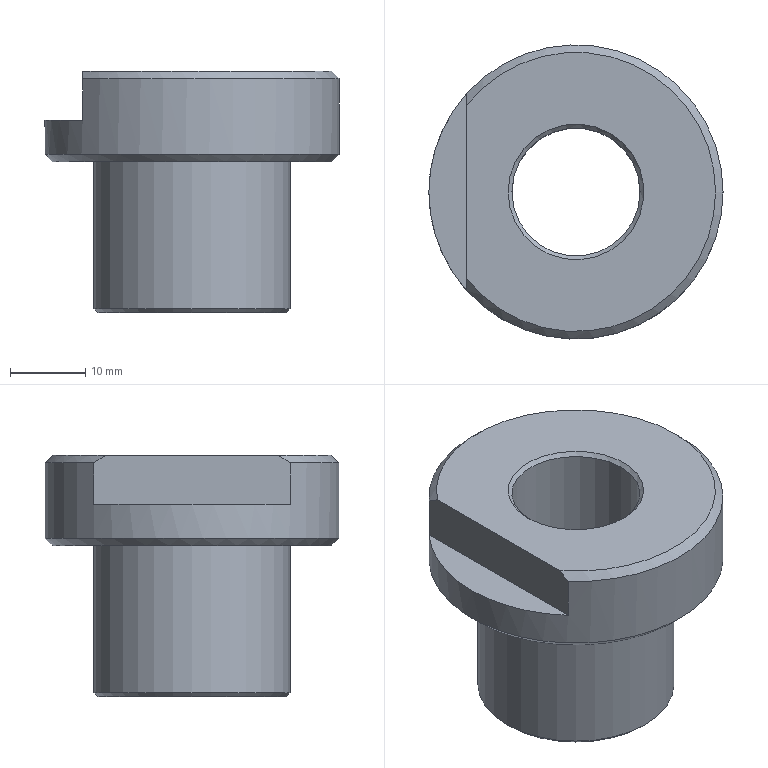Component | NX | DRILL_BUSH_2 | 1 solid | 13 faces | box 39 x 39 x 32 mm | volume 16979 mm3 | plane 5 | cone 5 | cylinder 3 | commonest cylinder face diameters 26 x1 39 x1 17 x1
STEP:
#1=CARTESIAN_POINT('',(0.,0.,0.));
#2=DIRECTION('',(0.,0.,1.));
#3=DIRECTION('',(1.,0.,0.));
#4=AXIS2_PLACEMENT_3D('',#1,#2,#3);
#5=CARTESIAN_POINT('',(99.,0.,190.));
#6=VERTEX_POINT('',#5);
#7=CARTESIAN_POINT('',(90.,0.,190.));
#8=DIRECTION('',(0.,0.,1.));
#9=DIRECTION('',(1.,0.,0.));
#10=AXIS2_PLACEMENT_3D('',#7,#8,#9);
#11=CIRCLE('',#10,9.);
#12=CARTESIAN_POINT('',(90.,0.,190.));
#13=DIRECTION('',(0.,0.,-1.));
#14=DIRECTION('',(1.,0.,0.));
#15=AXIS2_PLACEMENT_3D('',#12,#13,#14);
#16=PLANE('',#15);
#17=CARTESIAN_POINT('',(9.,0.));
#18=CARTESIAN_POINT('',(9.,-15.588));
#19=CARTESIAN_POINT('',(-4.5,-7.794));
#20=CARTESIAN_POINT('',(-18.,-0.));
#21=CARTESIAN_POINT('',(-4.5,7.794));
#22=CARTESIAN_POINT('',(9.,15.588));
#23=CARTESIAN_POINT('',(9.,0.));
#24=(BOUNDED_CURVE()B_SPLINE_CURVE(2,(#17,#18,#19,#20,#21,#22,#23),.UNSPECIFIED.,.T.,.F.)B_SPLINE_CURVE_WITH_KNOTS((1,2,2,2,2,1),(-2.094,0.,2.094,4.189,6.283,8.378),.UNSPECIFIED.)CURVE()GEOMETRIC_REPRESENTATION_ITEM()RATIONAL_B_SPLINE_CURVE((1.,0.5,1.,0.5,1.,0.5,1.))REPRESENTATION_ITEM(''));
#25=(GEOMETRIC_REPRESENTATION_CONTEXT(2)PARAMETRIC_REPRESENTATION_CONTEXT()REPRESENTATION_CONTEXT('',''));
#26=DEFINITIONAL_REPRESENTATION('',(#24),#25);
#27=PCURVE('',#16,#26);
#28=CARTESIAN_POINT('',(90.,0.,190.5));
#29=DIRECTION('',(0.,0.,-1.));
#30=DIRECTION('',(1.,0.,0.));
#31=AXIS2_PLACEMENT_3D('',#28,#29,#30);
#32=CONICAL_SURFACE('',#31,8.5,0.7854);
#33=CARTESIAN_POINT('',(6.283,0.5));
#34=DIRECTION('',(-1.,0.));
#35=VECTOR('',#34,1.);
#36=LINE('',#33,#35);
#37=(GEOMETRIC_REPRESENTATION_CONTEXT(2)PARAMETRIC_REPRESENTATION_CONTEXT()REPRESENTATION_CONTEXT('',''));
#38=DEFINITIONAL_REPRESENTATION('',(#36),#37);
#39=PCURVE('',#32,#38);
#40=SURFACE_CURVE('',#11,(#27,#39),.PCURVE_S1.);
#41=EDGE_CURVE('',#6,#6,#40,.T.);
#42=ORIENTED_EDGE('',*,*,#41,.T.);
#43=EDGE_LOOP('',(#42));
#44=FACE_BOUND('',#43,.T.);
#45=CARTESIAN_POINT('',(102.5,0.,190.));
#46=VERTEX_POINT('',#45);
#47=CARTESIAN_POINT('',(90.,0.,190.));
#48=DIRECTION('',(0.,0.,-1.));
#49=DIRECTION('',(1.,0.,0.));
#50=AXIS2_PLACEMENT_3D('',#47,#48,#49);
#51=CIRCLE('',#50,12.5);
#52=CARTESIAN_POINT('',(0.,0.));
#53=DIRECTION('',(1.,0.));
#54=AXIS2_PLACEMENT_2D('',#52,#53);
#55=CIRCLE('',#54,12.5);
#56=(GEOMETRIC_REPRESENTATION_CONTEXT(2)PARAMETRIC_REPRESENTATION_CONTEXT()REPRESENTATION_CONTEXT('',''));
#57=DEFINITIONAL_REPRESENTATION('',(#55),#56);
#58=PCURVE('',#16,#57);
#59=CARTESIAN_POINT('',(90.,0.,190.5));
#60=DIRECTION('',(0.,0.,1.));
#61=DIRECTION('',(-1.,0.,0.));
#62=AXIS2_PLACEMENT_3D('',#59,#60,#61);
#63=CONICAL_SURFACE('',#62,13.,0.7854);
#64=CARTESIAN_POINT('',(9.425,-0.5));
#65=DIRECTION('',(-1.,0.));
#66=VECTOR('',#65,1.);
#67=LINE('',#64,#66);
#68=(GEOMETRIC_REPRESENTATION_CONTEXT(2)PARAMETRIC_REPRESENTATION_CONTEXT()REPRESENTATION_CONTEXT('',''));
#69=DEFINITIONAL_REPRESENTATION('',(#67),#68);
#70=PCURVE('',#63,#69);
#71=SURFACE_CURVE('',#51,(#58,#70),.PCURVE_S1.);
#72=EDGE_CURVE('',#46,#46,#71,.T.);
#73=ORIENTED_EDGE('',*,*,#72,.T.);
#74=EDGE_LOOP('',(#73));
#75=FACE_BOUND('',#74,.T.);
#76=ADVANCED_FACE('',(#44,#75),#16,.T.);
#77=CARTESIAN_POINT('',(103.,0.,190.5));
#78=VERTEX_POINT('',#77);
#79=CARTESIAN_POINT('',(90.,0.,190.5));
#80=DIRECTION('',(0.,0.,1.));
#81=DIRECTION('',(1.,0.,0.));
#82=AXIS2_PLACEMENT_3D('',#79,#80,#81);
#83=CIRCLE('',#82,13.);
#84=CARTESIAN_POINT('',(90.,0.,190.));
#85=DIRECTION('',(0.,0.,1.));
#86=DIRECTION('',(-1.,0.,0.));
#87=AXIS2_PLACEMENT_3D('',#84,#85,#86);
#88=CYLINDRICAL_SURFACE('',#87,13.);
#89=CARTESIAN_POINT('',(3.142,0.5));
#90=DIRECTION('',(1.,0.));
#91=VECTOR('',#90,1.);
#92=LINE('',#89,#91);
#93=(GEOMETRIC_REPRESENTATION_CONTEXT(2)PARAMETRIC_REPRESENTATION_CONTEXT()REPRESENTATION_CONTEXT('',''));
#94=DEFINITIONAL_REPRESENTATION('',(#92),#93);
#95=PCURVE('',#88,#94);
#96=CARTESIAN_POINT('',(3.142,0.));
#97=DIRECTION('',(1.,0.));
#98=VECTOR('',#97,1.);
#99=LINE('',#96,#98);
#100=(GEOMETRIC_REPRESENTATION_CONTEXT(2)PARAMETRIC_REPRESENTATION_CONTEXT()REPRESENTATION_CONTEXT('',''));
#101=DEFINITIONAL_REPRESENTATION('',(#99),#100);
#102=PCURVE('',#63,#101);
#103=SURFACE_CURVE('',#83,(#95,#102),.PCURVE_S1.);
#104=EDGE_CURVE('',#78,#78,#103,.T.);
#105=ORIENTED_EDGE('',*,*,#104,.T.);
#106=CARTESIAN_POINT('',(103.,0.,210.));
#107=VERTEX_POINT('',#106);
#108=CARTESIAN_POINT('',(103.,0.,190.5));
#109=CARTESIAN_POINT('',(103.,0.,210.));
#110=B_SPLINE_CURVE_WITH_KNOTS('',1,(#108,#109),.UNSPECIFIED.,.F.,.F.,(2,2),(0.5,20.),.PIECEWISE_BEZIER_KNOTS.);
#111=CARTESIAN_POINT('',(9.425,0.));
#112=DIRECTION('',(0.,1.));
#113=VECTOR('',#112,1.);
#114=LINE('',#111,#113);
#115=(GEOMETRIC_REPRESENTATION_CONTEXT(2)PARAMETRIC_REPRESENTATION_CONTEXT()REPRESENTATION_CONTEXT('',''));
#116=DEFINITIONAL_REPRESENTATION('',(#114),#115);
#117=PCURVE('',#88,#116);
#118=CARTESIAN_POINT('',(3.142,0.));
#119=DIRECTION('',(0.,1.));
#120=VECTOR('',#119,1.);
#121=LINE('',#118,#120);
#122=(GEOMETRIC_REPRESENTATION_CONTEXT(2)PARAMETRIC_REPRESENTATION_CONTEXT()REPRESENTATION_CONTEXT('',''));
#123=DEFINITIONAL_REPRESENTATION('',(#121),#122);
#124=PCURVE('',#88,#123);
#125=SEAM_CURVE('',#110,(#117,#124),.PCURVE_S1.);
#126=EDGE_CURVE('',#78,#107,#125,.T.);
#127=ORIENTED_EDGE('',*,*,#126,.T.);
#128=CARTESIAN_POINT('',(90.,0.,210.));
#129=DIRECTION('',(0.,0.,1.));
#130=DIRECTION('',(1.,0.,0.));
#131=AXIS2_PLACEMENT_3D('',#128,#129,#130);
#132=CIRCLE('',#131,13.);
#133=CARTESIAN_POINT('',(3.142,20.));
#134=DIRECTION('',(1.,0.));
#135=VECTOR('',#134,1.);
#136=LINE('',#133,#135);
#137=(GEOMETRIC_REPRESENTATION_CONTEXT(2)PARAMETRIC_REPRESENTATION_CONTEXT()REPRESENTATION_CONTEXT('',''));
#138=DEFINITIONAL_REPRESENTATION('',(#136),#137);
#139=PCURVE('',#88,#138);
#140=CARTESIAN_POINT('',(90.,0.,210.));
#141=DIRECTION('',(0.,0.,-1.));
#142=DIRECTION('',(1.,0.,0.));
#143=AXIS2_PLACEMENT_3D('',#140,#141,#142);
#144=PLANE('',#143);
#145=CARTESIAN_POINT('',(13.,0.));
#146=CARTESIAN_POINT('',(13.,-22.517));
#147=CARTESIAN_POINT('',(-6.5,-11.258));
#148=CARTESIAN_POINT('',(-26.,-0.));
#149=CARTESIAN_POINT('',(-6.5,11.258));
#150=CARTESIAN_POINT('',(13.,22.517));
#151=CARTESIAN_POINT('',(13.,0.));
#152=(BOUNDED_CURVE()B_SPLINE_CURVE(2,(#145,#146,#147,#148,#149,#150,#151),.UNSPECIFIED.,.T.,.F.)B_SPLINE_CURVE_WITH_KNOTS((1,2,2,2,2,1),(-2.094,0.,2.094,4.189,6.283,8.378),.UNSPECIFIED.)CURVE()GEOMETRIC_REPRESENTATION_ITEM()RATIONAL_B_SPLINE_CURVE((1.,0.5,1.,0.5,1.,0.5,1.))REPRESENTATION_ITEM(''));
#153=(GEOMETRIC_REPRESENTATION_CONTEXT(2)PARAMETRIC_REPRESENTATION_CONTEXT()REPRESENTATION_CONTEXT('',''));
#154=DEFINITIONAL_REPRESENTATION('',(#152),#153);
#155=PCURVE('',#144,#154);
#156=SURFACE_CURVE('',#132,(#139,#155),.PCURVE_S1.);
#157=EDGE_CURVE('',#107,#107,#156,.T.);
#158=ORIENTED_EDGE('',*,*,#157,.F.);
#159=ORIENTED_EDGE('',*,*,#126,.F.);
#160=EDGE_LOOP('',(#105,#127,#158,#159));
#161=FACE_BOUND('',#160,.T.);
#162=ADVANCED_FACE('',(#161),#88,.T.);
#163=CARTESIAN_POINT('',(81.,0.,222.));
#164=VERTEX_POINT('',#163);
#165=CARTESIAN_POINT('',(90.,0.,222.));
#166=DIRECTION('',(0.,0.,-1.));
#167=DIRECTION('',(-1.,0.,0.));
#168=AXIS2_PLACEMENT_3D('',#165,#166,#167);
#169=CIRCLE('',#168,9.);
#170=CARTESIAN_POINT('',(90.,0.,222.));
#171=DIRECTION('',(0.,0.,1.));
#172=DIRECTION('',(-1.,0.,0.));
#173=AXIS2_PLACEMENT_3D('',#170,#171,#172);
#174=PLANE('',#173);
#175=CARTESIAN_POINT('',(9.,0.));
#176=CARTESIAN_POINT('',(9.,-15.588));
#177=CARTESIAN_POINT('',(-4.5,-7.794));
#178=CARTESIAN_POINT('',(-18.,-0.));
#179=CARTESIAN_POINT('',(-4.5,7.794));
#180=CARTESIAN_POINT('',(9.,15.588));
#181=CARTESIAN_POINT('',(9.,0.));
#182=(BOUNDED_CURVE()B_SPLINE_CURVE(2,(#175,#176,#177,#178,#179,#180,#181),.UNSPECIFIED.,.T.,.F.)B_SPLINE_CURVE_WITH_KNOTS((1,2,2,2,2,1),(-2.094,0.,2.094,4.189,6.283,8.378),.UNSPECIFIED.)CURVE()GEOMETRIC_REPRESENTATION_ITEM()RATIONAL_B_SPLINE_CURVE((1.,0.5,1.,0.5,1.,0.5,1.))REPRESENTATION_ITEM(''));
#183=(GEOMETRIC_REPRESENTATION_CONTEXT(2)PARAMETRIC_REPRESENTATION_CONTEXT()REPRESENTATION_CONTEXT('',''));
#184=DEFINITIONAL_REPRESENTATION('',(#182),#183);
#185=PCURVE('',#174,#184);
#186=CARTESIAN_POINT('',(90.,0.,222.));
#187=DIRECTION('',(0.,0.,1.));
#188=DIRECTION('',(-1.,0.,0.));
#189=AXIS2_PLACEMENT_3D('',#186,#187,#188);
#190=CONICAL_SURFACE('',#189,9.,0.7854);
#191=CARTESIAN_POINT('',(6.283,0.));
#192=DIRECTION('',(-1.,0.));
#193=VECTOR('',#192,1.);
#194=LINE('',#191,#193);
#195=(GEOMETRIC_REPRESENTATION_CONTEXT(2)PARAMETRIC_REPRESENTATION_CONTEXT()REPRESENTATION_CONTEXT('',''));
#196=DEFINITIONAL_REPRESENTATION('',(#194),#195);
#197=PCURVE('',#190,#196);
#198=SURFACE_CURVE('',#169,(#185,#197),.PCURVE_S1.);
#199=EDGE_CURVE('',#164,#164,#198,.T.);
#200=ORIENTED_EDGE('',*,*,#199,.T.);
#201=EDGE_LOOP('',(#200));
#202=FACE_BOUND('',#201,.T.);
#203=CARTESIAN_POINT('',(75.5,-11.489,222.));
#204=VERTEX_POINT('',#203);
#205=CARTESIAN_POINT('',(75.5,11.489,222.));
#206=VERTEX_POINT('',#205);
#207=CARTESIAN_POINT('',(75.5,-22.5,222.));
#208=DIRECTION('',(-0.,1.,0.));
#209=VECTOR('',#208,1.);
#210=LINE('',#207,#209);
#211=CARTESIAN_POINT('',(14.5,22.5));
#212=DIRECTION('',(0.,-1.));
#213=VECTOR('',#212,1.);
#214=LINE('',#211,#213);
#215=(GEOMETRIC_REPRESENTATION_CONTEXT(2)PARAMETRIC_REPRESENTATION_CONTEXT()REPRESENTATION_CONTEXT('',''));
#216=DEFINITIONAL_REPRESENTATION('',(#214),#215);
#217=PCURVE('',#174,#216);
#218=CARTESIAN_POINT('',(75.5,-22.5,215.5));
#219=DIRECTION('',(1.,0.,0.));
#220=DIRECTION('',(-0.,1.,0.));
#221=AXIS2_PLACEMENT_3D('',#218,#219,#220);
#222=PLANE('',#221);
#223=CARTESIAN_POINT('',(0.,6.5));
#224=DIRECTION('',(1.,0.));
#225=VECTOR('',#224,1.);
#226=LINE('',#223,#225);
#227=(GEOMETRIC_REPRESENTATION_CONTEXT(2)PARAMETRIC_REPRESENTATION_CONTEXT()REPRESENTATION_CONTEXT('',''));
#228=DEFINITIONAL_REPRESENTATION('',(#226),#227);
#229=PCURVE('',#222,#228);
#230=SURFACE_CURVE('',#210,(#217,#229),.PCURVE_S1.);
#231=EDGE_CURVE('',#204,#206,#230,.T.);
#232=ORIENTED_EDGE('',*,*,#231,.F.);
#233=CARTESIAN_POINT('',(90.,0.,222.));
#234=DIRECTION('',(0.,0.,1.));
#235=DIRECTION('',(-1.,0.,0.));
#236=AXIS2_PLACEMENT_3D('',#233,#234,#235);
#237=CIRCLE('',#236,18.5);
#238=CARTESIAN_POINT('',(0.,0.));
#239=DIRECTION('',(1.,0.));
#240=AXIS2_PLACEMENT_2D('',#238,#239);
#241=CIRCLE('',#240,18.5);
#242=(GEOMETRIC_REPRESENTATION_CONTEXT(2)PARAMETRIC_REPRESENTATION_CONTEXT()REPRESENTATION_CONTEXT('',''));
#243=DEFINITIONAL_REPRESENTATION('',(#241),#242);
#244=PCURVE('',#174,#243);
#245=CARTESIAN_POINT('',(90.,0.,221.));
#246=DIRECTION('',(0.,0.,-1.));
#247=DIRECTION('',(1.,0.,0.));
#248=AXIS2_PLACEMENT_3D('',#245,#246,#247);
#249=CONICAL_SURFACE('',#248,19.5,0.7854);
#250=CARTESIAN_POINT('',(3.142,-1.));
#251=DIRECTION('',(-1.,-0.));
#252=VECTOR('',#251,1.);
#253=LINE('',#250,#252);
#254=(GEOMETRIC_REPRESENTATION_CONTEXT(2)PARAMETRIC_REPRESENTATION_CONTEXT()REPRESENTATION_CONTEXT('',''));
#255=DEFINITIONAL_REPRESENTATION('',(#253),#254);
#256=PCURVE('',#249,#255);
#257=SURFACE_CURVE('',#237,(#244,#256),.PCURVE_S1.);
#258=EDGE_CURVE('',#204,#206,#257,.T.);
#259=ORIENTED_EDGE('',*,*,#258,.T.);
#260=EDGE_LOOP('',(#232,#259));
#261=FACE_BOUND('',#260,.T.);
#262=ADVANCED_FACE('',(#202,#261),#174,.T.);
#263=CARTESIAN_POINT('',(108.5,0.,210.));
#264=VERTEX_POINT('',#263);
#265=CARTESIAN_POINT('',(90.,0.,210.));
#266=DIRECTION('',(0.,0.,-1.));
#267=DIRECTION('',(1.,0.,0.));
#268=AXIS2_PLACEMENT_3D('',#265,#266,#267);
#269=CIRCLE('',#268,18.5);
#270=CARTESIAN_POINT('',(0.,0.));
#271=DIRECTION('',(1.,0.));
#272=AXIS2_PLACEMENT_2D('',#270,#271);
#273=CIRCLE('',#272,18.5);
#274=(GEOMETRIC_REPRESENTATION_CONTEXT(2)PARAMETRIC_REPRESENTATION_CONTEXT()REPRESENTATION_CONTEXT('',''));
#275=DEFINITIONAL_REPRESENTATION('',(#273),#274);
#276=PCURVE('',#144,#275);
#277=CARTESIAN_POINT('',(90.,0.,211.));
#278=DIRECTION('',(0.,0.,1.));
#279=DIRECTION('',(-1.,0.,0.));
#280=AXIS2_PLACEMENT_3D('',#277,#278,#279);
#281=CONICAL_SURFACE('',#280,19.5,0.7854);
#282=CARTESIAN_POINT('',(9.425,-1.));
#283=DIRECTION('',(-1.,0.));
#284=VECTOR('',#283,1.);
#285=LINE('',#282,#284);
#286=(GEOMETRIC_REPRESENTATION_CONTEXT(2)PARAMETRIC_REPRESENTATION_CONTEXT()REPRESENTATION_CONTEXT('',''));
#287=DEFINITIONAL_REPRESENTATION('',(#285),#286);
#288=PCURVE('',#281,#287);
#289=SURFACE_CURVE('',#269,(#276,#288),.PCURVE_S1.);
#290=EDGE_CURVE('',#264,#264,#289,.T.);
#291=ORIENTED_EDGE('',*,*,#290,.T.);
#292=EDGE_LOOP('',(#291));
#293=FACE_BOUND('',#292,.T.);
#294=ORIENTED_EDGE('',*,*,#157,.T.);
#295=EDGE_LOOP('',(#294));
#296=FACE_BOUND('',#295,.T.);
#297=ADVANCED_FACE('',(#293,#296),#144,.T.);
#298=CARTESIAN_POINT('',(109.5,0.,211.));
#299=VERTEX_POINT('',#298);
#300=CARTESIAN_POINT('',(75.5,13.038,211.));
#301=VERTEX_POINT('',#300);
#302=CARTESIAN_POINT('',(90.,0.,211.));
#303=DIRECTION('',(0.,0.,1.));
#304=DIRECTION('',(1.,0.,0.));
#305=AXIS2_PLACEMENT_3D('',#302,#303,#304);
#306=CIRCLE('',#305,19.5);
#307=CARTESIAN_POINT('',(90.,0.,210.));
#308=DIRECTION('',(0.,0.,1.));
#309=DIRECTION('',(-1.,0.,0.));
#310=AXIS2_PLACEMENT_3D('',#307,#308,#309);
#311=CYLINDRICAL_SURFACE('',#310,19.5);
#312=CARTESIAN_POINT('',(9.425,1.));
#313=DIRECTION('',(1.,0.));
#314=VECTOR('',#313,1.);
#315=LINE('',#312,#314);
#316=(GEOMETRIC_REPRESENTATION_CONTEXT(2)PARAMETRIC_REPRESENTATION_CONTEXT()REPRESENTATION_CONTEXT('',''));
#317=DEFINITIONAL_REPRESENTATION('',(#315),#316);
#318=PCURVE('',#311,#317);
#319=CARTESIAN_POINT('',(3.142,0.));
#320=DIRECTION('',(1.,0.));
#321=VECTOR('',#320,1.);
#322=LINE('',#319,#321);
#323=(GEOMETRIC_REPRESENTATION_CONTEXT(2)PARAMETRIC_REPRESENTATION_CONTEXT()REPRESENTATION_CONTEXT('',''));
#324=DEFINITIONAL_REPRESENTATION('',(#322),#323);
#325=PCURVE('',#281,#324);
#326=SURFACE_CURVE('',#306,(#318,#325),.PCURVE_S1.);
#327=EDGE_CURVE('',#299,#301,#326,.T.);
#328=ORIENTED_EDGE('',*,*,#327,.T.);
#329=CARTESIAN_POINT('',(75.5,13.038,215.5));
#330=VERTEX_POINT('',#329);
#331=CARTESIAN_POINT('',(75.5,13.038,211.));
#332=CARTESIAN_POINT('',(75.5,13.038,215.5));
#333=B_SPLINE_CURVE_WITH_KNOTS('',1,(#331,#332),.UNSPECIFIED.,.F.,.F.,(2,2),(1.,5.5),.PIECEWISE_BEZIER_KNOTS.);
#334=CARTESIAN_POINT('',(11.834,0.));
#335=DIRECTION('',(0.,1.));
#336=VECTOR('',#335,1.);
#337=LINE('',#334,#336);
#338=(GEOMETRIC_REPRESENTATION_CONTEXT(2)PARAMETRIC_REPRESENTATION_CONTEXT()REPRESENTATION_CONTEXT('',''));
#339=DEFINITIONAL_REPRESENTATION('',(#337),#338);
#340=PCURVE('',#311,#339);
#341=CARTESIAN_POINT('',(5.551,0.));
#342=DIRECTION('',(0.,1.));
#343=VECTOR('',#342,1.);
#344=LINE('',#341,#343);
#345=(GEOMETRIC_REPRESENTATION_CONTEXT(2)PARAMETRIC_REPRESENTATION_CONTEXT()REPRESENTATION_CONTEXT('',''));
#346=DEFINITIONAL_REPRESENTATION('',(#344),#345);
#347=PCURVE('',#311,#346);
#348=SEAM_CURVE('',#333,(#340,#347),.PCURVE_S1.);
#349=EDGE_CURVE('',#301,#330,#348,.T.);
#350=ORIENTED_EDGE('',*,*,#349,.T.);
#351=CARTESIAN_POINT('',(75.5,13.038,221.));
#352=VERTEX_POINT('',#351);
#353=CARTESIAN_POINT('',(75.5,13.038,210.));
#354=DIRECTION('',(0.,0.,-1.));
#355=VECTOR('',#354,1.);
#356=LINE('',#353,#355);
#357=CARTESIAN_POINT('',(11.834,0.));
#358=DIRECTION('',(0.,-1.));
#359=VECTOR('',#358,1.);
#360=LINE('',#357,#359);
#361=(GEOMETRIC_REPRESENTATION_CONTEXT(2)PARAMETRIC_REPRESENTATION_CONTEXT()REPRESENTATION_CONTEXT('',''));
#362=DEFINITIONAL_REPRESENTATION('',(#360),#361);
#363=PCURVE('',#311,#362);
#364=CARTESIAN_POINT('',(35.538,-5.5));
#365=DIRECTION('',(0.,-1.));
#366=VECTOR('',#365,1.);
#367=LINE('',#364,#366);
#368=(GEOMETRIC_REPRESENTATION_CONTEXT(2)PARAMETRIC_REPRESENTATION_CONTEXT()REPRESENTATION_CONTEXT('',''));
#369=DEFINITIONAL_REPRESENTATION('',(#367),#368);
#370=PCURVE('',#222,#369);
#371=SURFACE_CURVE('',#356,(#363,#370),.PCURVE_S1.);
#372=EDGE_CURVE('',#352,#330,#371,.T.);
#373=ORIENTED_EDGE('',*,*,#372,.F.);
#374=CARTESIAN_POINT('',(75.5,-13.038,221.));
#375=VERTEX_POINT('',#374);
#376=CARTESIAN_POINT('',(90.,0.,221.));
#377=DIRECTION('',(0.,0.,-1.));
#378=DIRECTION('',(-1.,0.,0.));
#379=AXIS2_PLACEMENT_3D('',#376,#377,#378);
#380=CIRCLE('',#379,19.5);
#381=CARTESIAN_POINT('',(12.566,11.));
#382=DIRECTION('',(-1.,0.));
#383=VECTOR('',#382,1.);
#384=LINE('',#381,#383);
#385=(GEOMETRIC_REPRESENTATION_CONTEXT(2)PARAMETRIC_REPRESENTATION_CONTEXT()REPRESENTATION_CONTEXT('',''));
#386=DEFINITIONAL_REPRESENTATION('',(#384),#385);
#387=PCURVE('',#311,#386);
#388=CARTESIAN_POINT('',(-3.142,-0.));
#389=DIRECTION('',(1.,0.));
#390=VECTOR('',#389,1.);
#391=LINE('',#388,#390);
#392=(GEOMETRIC_REPRESENTATION_CONTEXT(2)PARAMETRIC_REPRESENTATION_CONTEXT()REPRESENTATION_CONTEXT('',''));
#393=DEFINITIONAL_REPRESENTATION('',(#391),#392);
#394=PCURVE('',#249,#393);
#395=SURFACE_CURVE('',#380,(#387,#394),.PCURVE_S1.);
#396=EDGE_CURVE('',#352,#375,#395,.T.);
#397=ORIENTED_EDGE('',*,*,#396,.T.);
#398=CARTESIAN_POINT('',(75.5,-13.038,215.5));
#399=VERTEX_POINT('',#398);
#400=CARTESIAN_POINT('',(75.5,-13.038,210.));
#401=DIRECTION('',(0.,0.,1.));
#402=VECTOR('',#401,1.);
#403=LINE('',#400,#402);
#404=CARTESIAN_POINT('',(7.016,0.));
#405=DIRECTION('',(0.,1.));
#406=VECTOR('',#405,1.);
#407=LINE('',#404,#406);
#408=(GEOMETRIC_REPRESENTATION_CONTEXT(2)PARAMETRIC_REPRESENTATION_CONTEXT()REPRESENTATION_CONTEXT('',''));
#409=DEFINITIONAL_REPRESENTATION('',(#407),#408);
#410=PCURVE('',#311,#409);
#411=CARTESIAN_POINT('',(9.462,-5.5));
#412=DIRECTION('',(0.,1.));
#413=VECTOR('',#412,1.);
#414=LINE('',#411,#413);
#415=(GEOMETRIC_REPRESENTATION_CONTEXT(2)PARAMETRIC_REPRESENTATION_CONTEXT()REPRESENTATION_CONTEXT('',''));
#416=DEFINITIONAL_REPRESENTATION('',(#414),#415);
#417=PCURVE('',#222,#416);
#418=SURFACE_CURVE('',#403,(#410,#417),.PCURVE_S1.);
#419=EDGE_CURVE('',#399,#375,#418,.T.);
#420=ORIENTED_EDGE('',*,*,#419,.F.);
#421=CARTESIAN_POINT('',(90.,0.,215.5));
#422=DIRECTION('',(0.,0.,-1.));
#423=DIRECTION('',(-1.,0.,0.));
#424=AXIS2_PLACEMENT_3D('',#421,#422,#423);
#425=CIRCLE('',#424,19.5);
#426=CARTESIAN_POINT('',(12.566,5.5));
#427=DIRECTION('',(-1.,0.));
#428=VECTOR('',#427,1.);
#429=LINE('',#426,#428);
#430=(GEOMETRIC_REPRESENTATION_CONTEXT(2)PARAMETRIC_REPRESENTATION_CONTEXT()REPRESENTATION_CONTEXT('',''));
#431=DEFINITIONAL_REPRESENTATION('',(#429),#430);
#432=PCURVE('',#311,#431);
#433=CARTESIAN_POINT('',(90.,0.,215.5));
#434=DIRECTION('',(0.,0.,1.));
#435=DIRECTION('',(-1.,0.,0.));
#436=AXIS2_PLACEMENT_3D('',#433,#434,#435);
#437=PLANE('',#436);
#438=CARTESIAN_POINT('',(19.5,0.));
#439=CARTESIAN_POINT('',(19.5,-33.775));
#440=CARTESIAN_POINT('',(-9.75,-16.887));
#441=CARTESIAN_POINT('',(-39.,-0.));
#442=CARTESIAN_POINT('',(-9.75,16.887));
#443=CARTESIAN_POINT('',(19.5,33.775));
#444=CARTESIAN_POINT('',(19.5,0.));
#445=(BOUNDED_CURVE()B_SPLINE_CURVE(2,(#438,#439,#440,#441,#442,#443,#444),.UNSPECIFIED.,.T.,.F.)B_SPLINE_CURVE_WITH_KNOTS((1,2,2,2,2,1),(-2.094,0.,2.094,4.189,6.283,8.378),.UNSPECIFIED.)CURVE()GEOMETRIC_REPRESENTATION_ITEM()RATIONAL_B_SPLINE_CURVE((1.,0.5,1.,0.5,1.,0.5,1.))REPRESENTATION_ITEM(''));
#446=(GEOMETRIC_REPRESENTATION_CONTEXT(2)PARAMETRIC_REPRESENTATION_CONTEXT()REPRESENTATION_CONTEXT('',''));
#447=DEFINITIONAL_REPRESENTATION('',(#445),#446);
#448=PCURVE('',#437,#447);
#449=SURFACE_CURVE('',#425,(#432,#448),.PCURVE_S1.);
#450=EDGE_CURVE('',#399,#330,#449,.T.);
#451=ORIENTED_EDGE('',*,*,#450,.T.);
#452=ORIENTED_EDGE('',*,*,#349,.F.);
#453=CARTESIAN_POINT('',(90.,0.,211.));
#454=DIRECTION('',(0.,0.,1.));
#455=DIRECTION('',(1.,0.,0.));
#456=AXIS2_PLACEMENT_3D('',#453,#454,#455);
#457=CIRCLE('',#456,19.5);
#458=CARTESIAN_POINT('',(3.142,1.));
#459=DIRECTION('',(1.,0.));
#460=VECTOR('',#459,1.);
#461=LINE('',#458,#460);
#462=(GEOMETRIC_REPRESENTATION_CONTEXT(2)PARAMETRIC_REPRESENTATION_CONTEXT()REPRESENTATION_CONTEXT('',''));
#463=DEFINITIONAL_REPRESENTATION('',(#461),#462);
#464=PCURVE('',#311,#463);
#465=CARTESIAN_POINT('',(3.142,0.));
#466=DIRECTION('',(1.,0.));
#467=VECTOR('',#466,1.);
#468=LINE('',#465,#467);
#469=(GEOMETRIC_REPRESENTATION_CONTEXT(2)PARAMETRIC_REPRESENTATION_CONTEXT()REPRESENTATION_CONTEXT('',''));
#470=DEFINITIONAL_REPRESENTATION('',(#468),#469);
#471=PCURVE('',#281,#470);
#472=SURFACE_CURVE('',#457,(#464,#471),.PCURVE_S1.);
#473=EDGE_CURVE('',#301,#299,#472,.T.);
#474=ORIENTED_EDGE('',*,*,#473,.T.);
#475=EDGE_LOOP('',(#328,#350,#373,#397,#420,#451,#452,#474));
#476=FACE_BOUND('',#475,.T.);
#477=ADVANCED_FACE('',(#476),#311,.T.);
#478=ORIENTED_EDGE('',*,*,#419,.T.);
#479=CARTESIAN_POINT('',(75.5,-13.038,221.));
#480=CARTESIAN_POINT('',(75.5,-12.527,221.342));
#481=CARTESIAN_POINT('',(75.5,-12.011,221.676));
#482=CARTESIAN_POINT('',(75.5,-11.489,222.));
#483=B_SPLINE_CURVE_WITH_KNOTS('',3,(#479,#480,#481,#482),.UNSPECIFIED.,.F.,.F.,(4,4),(0.,1.),.PIECEWISE_BEZIER_KNOTS.);
#484=CARTESIAN_POINT('',(9.462,5.5));
#485=CARTESIAN_POINT('',(9.973,5.842));
#486=CARTESIAN_POINT('',(10.489,6.176));
#487=CARTESIAN_POINT('',(11.011,6.5));
#488=B_SPLINE_CURVE_WITH_KNOTS('',3,(#484,#485,#486,#487),.UNSPECIFIED.,.F.,.F.,(4,4),(0.,1.),.PIECEWISE_BEZIER_KNOTS.);
#489=(GEOMETRIC_REPRESENTATION_CONTEXT(2)PARAMETRIC_REPRESENTATION_CONTEXT()REPRESENTATION_CONTEXT('',''));
#490=DEFINITIONAL_REPRESENTATION('',(#488),#489);
#491=PCURVE('',#222,#490);
#492=CARTESIAN_POINT('',(2.409,0.));
#493=CARTESIAN_POINT('',(2.472,-1.));
#494=B_SPLINE_CURVE_WITH_KNOTS('',1,(#492,#493),.UNSPECIFIED.,.F.,.F.,(2,2),(0.,1.),.PIECEWISE_BEZIER_KNOTS.);
#495=(GEOMETRIC_REPRESENTATION_CONTEXT(2)PARAMETRIC_REPRESENTATION_CONTEXT()REPRESENTATION_CONTEXT('',''));
#496=DEFINITIONAL_REPRESENTATION('',(#494),#495);
#497=PCURVE('',#249,#496);
#498=SURFACE_CURVE('',#483,(#491,#497),.PCURVE_S1.);
#499=EDGE_CURVE('',#375,#204,#498,.T.);
#500=ORIENTED_EDGE('',*,*,#499,.T.);
#501=ORIENTED_EDGE('',*,*,#231,.T.);
#502=CARTESIAN_POINT('',(75.5,11.489,222.));
#503=CARTESIAN_POINT('',(75.5,12.011,221.676));
#504=CARTESIAN_POINT('',(75.5,12.527,221.342));
#505=CARTESIAN_POINT('',(75.5,13.038,221.));
#506=B_SPLINE_CURVE_WITH_KNOTS('',3,(#502,#503,#504,#505),.UNSPECIFIED.,.F.,.F.,(4,4),(0.,1.),.PIECEWISE_BEZIER_KNOTS.);
#507=CARTESIAN_POINT('',(33.989,6.5));
#508=CARTESIAN_POINT('',(34.511,6.176));
#509=CARTESIAN_POINT('',(35.027,5.842));
#510=CARTESIAN_POINT('',(35.538,5.5));
#511=B_SPLINE_CURVE_WITH_KNOTS('',3,(#507,#508,#509,#510),.UNSPECIFIED.,.F.,.F.,(4,4),(0.,1.),.PIECEWISE_BEZIER_KNOTS.);
#512=(GEOMETRIC_REPRESENTATION_CONTEXT(2)PARAMETRIC_REPRESENTATION_CONTEXT()REPRESENTATION_CONTEXT('',''));
#513=DEFINITIONAL_REPRESENTATION('',(#511),#512);
#514=PCURVE('',#222,#513);
#515=CARTESIAN_POINT('',(-2.472,-1.));
#516=CARTESIAN_POINT('',(-2.409,-0.));
#517=B_SPLINE_CURVE_WITH_KNOTS('',1,(#515,#516),.UNSPECIFIED.,.F.,.F.,(2,2),(0.,1.),.PIECEWISE_BEZIER_KNOTS.);
#518=(GEOMETRIC_REPRESENTATION_CONTEXT(2)PARAMETRIC_REPRESENTATION_CONTEXT()REPRESENTATION_CONTEXT('',''));
#519=DEFINITIONAL_REPRESENTATION('',(#517),#518);
#520=PCURVE('',#249,#519);
#521=SURFACE_CURVE('',#506,(#514,#520),.PCURVE_S1.);
#522=EDGE_CURVE('',#206,#352,#521,.T.);
#523=ORIENTED_EDGE('',*,*,#522,.T.);
#524=ORIENTED_EDGE('',*,*,#372,.T.);
#525=CARTESIAN_POINT('',(75.5,-22.5,215.5));
#526=DIRECTION('',(0.,-1.,0.));
#527=VECTOR('',#526,1.);
#528=LINE('',#525,#527);
#529=CARTESIAN_POINT('',(0.,0.));
#530=DIRECTION('',(-1.,0.));
#531=VECTOR('',#530,1.);
#532=LINE('',#529,#531);
#533=(GEOMETRIC_REPRESENTATION_CONTEXT(2)PARAMETRIC_REPRESENTATION_CONTEXT()REPRESENTATION_CONTEXT('',''));
#534=DEFINITIONAL_REPRESENTATION('',(#532),#533);
#535=PCURVE('',#222,#534);
#536=CARTESIAN_POINT('',(14.5,22.5));
#537=DIRECTION('',(-0.,1.));
#538=VECTOR('',#537,1.);
#539=LINE('',#536,#538);
#540=(GEOMETRIC_REPRESENTATION_CONTEXT(2)PARAMETRIC_REPRESENTATION_CONTEXT()REPRESENTATION_CONTEXT('',''));
#541=DEFINITIONAL_REPRESENTATION('',(#539),#540);
#542=PCURVE('',#437,#541);
#543=SURFACE_CURVE('',#528,(#535,#542),.PCURVE_S1.);
#544=EDGE_CURVE('',#330,#399,#543,.T.);
#545=ORIENTED_EDGE('',*,*,#544,.T.);
#546=EDGE_LOOP('',(#478,#500,#501,#523,#524,#545));
#547=FACE_BOUND('',#546,.T.);
#548=ADVANCED_FACE('',(#547),#222,.F.);
#549=ORIENTED_EDGE('',*,*,#544,.F.);
#550=ORIENTED_EDGE('',*,*,#450,.F.);
#551=EDGE_LOOP('',(#549,#550));
#552=FACE_BOUND('',#551,.T.);
#553=ADVANCED_FACE('',(#552),#437,.T.);
#554=CARTESIAN_POINT('',(98.5,0.,190.5));
#555=VERTEX_POINT('',#554);
#556=CARTESIAN_POINT('',(90.,0.,190.5));
#557=DIRECTION('',(0.,0.,-1.));
#558=DIRECTION('',(1.,0.,0.));
#559=AXIS2_PLACEMENT_3D('',#556,#557,#558);
#560=CIRCLE('',#559,8.5);
#561=CARTESIAN_POINT('',(90.,0.,222.));
#562=DIRECTION('',(0.,0.,-1.));
#563=DIRECTION('',(1.,0.,0.));
#564=AXIS2_PLACEMENT_3D('',#561,#562,#563);
#565=CYLINDRICAL_SURFACE('',#564,8.5);
#566=CARTESIAN_POINT('',(0.,31.5));
#567=DIRECTION('',(1.,0.));
#568=VECTOR('',#567,1.);
#569=LINE('',#566,#568);
#570=(GEOMETRIC_REPRESENTATION_CONTEXT(2)PARAMETRIC_REPRESENTATION_CONTEXT()REPRESENTATION_CONTEXT('',''));
#571=DEFINITIONAL_REPRESENTATION('',(#569),#570);
#572=PCURVE('',#565,#571);
#573=CARTESIAN_POINT('',(0.,0.));
#574=DIRECTION('',(1.,0.));
#575=VECTOR('',#574,1.);
#576=LINE('',#573,#575);
#577=(GEOMETRIC_REPRESENTATION_CONTEXT(2)PARAMETRIC_REPRESENTATION_CONTEXT()REPRESENTATION_CONTEXT('',''));
#578=DEFINITIONAL_REPRESENTATION('',(#576),#577);
#579=PCURVE('',#32,#578);
#580=SURFACE_CURVE('',#560,(#572,#579),.PCURVE_S1.);
#581=EDGE_CURVE('',#555,#555,#580,.T.);
#582=ORIENTED_EDGE('',*,*,#581,.F.);
#583=CARTESIAN_POINT('',(98.5,0.,221.5));
#584=VERTEX_POINT('',#583);
#585=CARTESIAN_POINT('',(98.5,0.,221.5));
#586=CARTESIAN_POINT('',(98.5,0.,190.5));
#587=B_SPLINE_CURVE_WITH_KNOTS('',1,(#585,#586),.UNSPECIFIED.,.F.,.F.,(2,2),(0.5,31.5),.PIECEWISE_BEZIER_KNOTS.);
#588=CARTESIAN_POINT('',(0.,0.));
#589=DIRECTION('',(0.,1.));
#590=VECTOR('',#589,1.);
#591=LINE('',#588,#590);
#592=(GEOMETRIC_REPRESENTATION_CONTEXT(2)PARAMETRIC_REPRESENTATION_CONTEXT()REPRESENTATION_CONTEXT('',''));
#593=DEFINITIONAL_REPRESENTATION('',(#591),#592);
#594=PCURVE('',#565,#593);
#595=CARTESIAN_POINT('',(6.283,0.));
#596=DIRECTION('',(0.,1.));
#597=VECTOR('',#596,1.);
#598=LINE('',#595,#597);
#599=(GEOMETRIC_REPRESENTATION_CONTEXT(2)PARAMETRIC_REPRESENTATION_CONTEXT()REPRESENTATION_CONTEXT('',''));
#600=DEFINITIONAL_REPRESENTATION('',(#598),#599);
#601=PCURVE('',#565,#600);
#602=SEAM_CURVE('',#587,(#594,#601),.PCURVE_S1.);
#603=EDGE_CURVE('',#584,#555,#602,.T.);
#604=ORIENTED_EDGE('',*,*,#603,.F.);
#605=CARTESIAN_POINT('',(81.5,0.,221.5));
#606=VERTEX_POINT('',#605);
#607=CARTESIAN_POINT('',(90.,0.,221.5));
#608=DIRECTION('',(0.,0.,1.));
#609=DIRECTION('',(-1.,0.,0.));
#610=AXIS2_PLACEMENT_3D('',#607,#608,#609);
#611=CIRCLE('',#610,8.5);
#612=CARTESIAN_POINT('',(3.142,0.5));
#613=DIRECTION('',(-1.,0.));
#614=VECTOR('',#613,1.);
#615=LINE('',#612,#614);
#616=(GEOMETRIC_REPRESENTATION_CONTEXT(2)PARAMETRIC_REPRESENTATION_CONTEXT()REPRESENTATION_CONTEXT('',''));
#617=DEFINITIONAL_REPRESENTATION('',(#615),#616);
#618=PCURVE('',#565,#617);
#619=CARTESIAN_POINT('',(0.,-0.5));
#620=DIRECTION('',(1.,0.));
#621=VECTOR('',#620,1.);
#622=LINE('',#619,#621);
#623=(GEOMETRIC_REPRESENTATION_CONTEXT(2)PARAMETRIC_REPRESENTATION_CONTEXT()REPRESENTATION_CONTEXT('',''));
#624=DEFINITIONAL_REPRESENTATION('',(#622),#623);
#625=PCURVE('',#190,#624);
#626=SURFACE_CURVE('',#611,(#618,#625),.PCURVE_S1.);
#627=EDGE_CURVE('',#606,#584,#626,.T.);
#628=ORIENTED_EDGE('',*,*,#627,.F.);
#629=CARTESIAN_POINT('',(90.,0.,221.5));
#630=DIRECTION('',(0.,0.,1.));
#631=DIRECTION('',(-1.,0.,0.));
#632=AXIS2_PLACEMENT_3D('',#629,#630,#631);
#633=CIRCLE('',#632,8.5);
#634=CARTESIAN_POINT('',(9.425,0.5));
#635=DIRECTION('',(-1.,0.));
#636=VECTOR('',#635,1.);
#637=LINE('',#634,#636);
#638=(GEOMETRIC_REPRESENTATION_CONTEXT(2)PARAMETRIC_REPRESENTATION_CONTEXT()REPRESENTATION_CONTEXT('',''));
#639=DEFINITIONAL_REPRESENTATION('',(#637),#638);
#640=PCURVE('',#565,#639);
#641=CARTESIAN_POINT('',(0.,-0.5));
#642=DIRECTION('',(1.,0.));
#643=VECTOR('',#642,1.);
#644=LINE('',#641,#643);
#645=(GEOMETRIC_REPRESENTATION_CONTEXT(2)PARAMETRIC_REPRESENTATION_CONTEXT()REPRESENTATION_CONTEXT('',''));
#646=DEFINITIONAL_REPRESENTATION('',(#644),#645);
#647=PCURVE('',#190,#646);
#648=SURFACE_CURVE('',#633,(#640,#647),.PCURVE_S1.);
#649=EDGE_CURVE('',#584,#606,#648,.T.);
#650=ORIENTED_EDGE('',*,*,#649,.F.);
#651=ORIENTED_EDGE('',*,*,#603,.T.);
#652=EDGE_LOOP('',(#582,#604,#628,#650,#651));
#653=FACE_BOUND('',#652,.F.);
#654=ADVANCED_FACE('',(#653),#565,.F.);
#655=ORIENTED_EDGE('',*,*,#290,.F.);
#656=CARTESIAN_POINT('',(108.5,0.,210.));
#657=CARTESIAN_POINT('',(109.5,0.,211.));
#658=B_SPLINE_CURVE_WITH_KNOTS('',1,(#656,#657),.UNSPECIFIED.,.F.,.F.,(2,2),(-1.414,0.),.PIECEWISE_BEZIER_KNOTS.);
#659=CARTESIAN_POINT('',(9.425,0.));
#660=DIRECTION('',(0.,1.));
#661=VECTOR('',#660,1.);
#662=LINE('',#659,#661);
#663=(GEOMETRIC_REPRESENTATION_CONTEXT(2)PARAMETRIC_REPRESENTATION_CONTEXT()REPRESENTATION_CONTEXT('',''));
#664=DEFINITIONAL_REPRESENTATION('',(#662),#663);
#665=PCURVE('',#281,#664);
#666=CARTESIAN_POINT('',(3.142,0.));
#667=DIRECTION('',(0.,1.));
#668=VECTOR('',#667,1.);
#669=LINE('',#666,#668);
#670=(GEOMETRIC_REPRESENTATION_CONTEXT(2)PARAMETRIC_REPRESENTATION_CONTEXT()REPRESENTATION_CONTEXT('',''));
#671=DEFINITIONAL_REPRESENTATION('',(#669),#670);
#672=PCURVE('',#281,#671);
#673=SEAM_CURVE('',#658,(#665,#672),.PCURVE_S1.);
#674=EDGE_CURVE('',#264,#299,#673,.T.);
#675=ORIENTED_EDGE('',*,*,#674,.T.);
#676=ORIENTED_EDGE('',*,*,#473,.F.);
#677=ORIENTED_EDGE('',*,*,#327,.F.);
#678=ORIENTED_EDGE('',*,*,#674,.F.);
#679=EDGE_LOOP('',(#655,#675,#676,#677,#678));
#680=FACE_BOUND('',#679,.T.);
#681=ADVANCED_FACE('',(#680),#281,.T.);
#682=ORIENTED_EDGE('',*,*,#522,.F.);
#683=ORIENTED_EDGE('',*,*,#258,.F.);
#684=ORIENTED_EDGE('',*,*,#499,.F.);
#685=ORIENTED_EDGE('',*,*,#396,.F.);
#686=EDGE_LOOP('',(#682,#683,#684,#685));
#687=FACE_BOUND('',#686,.T.);
#688=ADVANCED_FACE('',(#687),#249,.T.);
#689=ORIENTED_EDGE('',*,*,#41,.T.);
#690=CARTESIAN_POINT('',(98.5,0.,190.5));
#691=CARTESIAN_POINT('',(99.,0.,190.));
#692=B_SPLINE_CURVE_WITH_KNOTS('',1,(#690,#691),.UNSPECIFIED.,.F.,.F.,(2,2),(0.,0.7071),.PIECEWISE_BEZIER_KNOTS.);
#693=CARTESIAN_POINT('',(0.,0.));
#694=DIRECTION('',(0.,1.));
#695=VECTOR('',#694,1.);
#696=LINE('',#693,#695);
#697=(GEOMETRIC_REPRESENTATION_CONTEXT(2)PARAMETRIC_REPRESENTATION_CONTEXT()REPRESENTATION_CONTEXT('',''));
#698=DEFINITIONAL_REPRESENTATION('',(#696),#697);
#699=PCURVE('',#32,#698);
#700=CARTESIAN_POINT('',(6.283,0.));
#701=DIRECTION('',(0.,1.));
#702=VECTOR('',#701,1.);
#703=LINE('',#700,#702);
#704=(GEOMETRIC_REPRESENTATION_CONTEXT(2)PARAMETRIC_REPRESENTATION_CONTEXT()REPRESENTATION_CONTEXT('',''));
#705=DEFINITIONAL_REPRESENTATION('',(#703),#704);
#706=PCURVE('',#32,#705);
#707=SEAM_CURVE('',#692,(#699,#706),.PCURVE_S1.);
#708=EDGE_CURVE('',#555,#6,#707,.T.);
#709=ORIENTED_EDGE('',*,*,#708,.F.);
#710=ORIENTED_EDGE('',*,*,#581,.T.);
#711=ORIENTED_EDGE('',*,*,#708,.T.);
#712=EDGE_LOOP('',(#689,#709,#710,#711));
#713=FACE_BOUND('',#712,.F.);
#714=ADVANCED_FACE('',(#713),#32,.F.);
#715=ORIENTED_EDGE('',*,*,#72,.F.);
#716=CARTESIAN_POINT('',(102.5,0.,190.));
#717=CARTESIAN_POINT('',(103.,0.,190.5));
#718=B_SPLINE_CURVE_WITH_KNOTS('',1,(#716,#717),.UNSPECIFIED.,.F.,.F.,(2,2),(-0.7071,0.),.PIECEWISE_BEZIER_KNOTS.);
#719=CARTESIAN_POINT('',(9.425,0.));
#720=DIRECTION('',(0.,1.));
#721=VECTOR('',#720,1.);
#722=LINE('',#719,#721);
#723=(GEOMETRIC_REPRESENTATION_CONTEXT(2)PARAMETRIC_REPRESENTATION_CONTEXT()REPRESENTATION_CONTEXT('',''));
#724=DEFINITIONAL_REPRESENTATION('',(#722),#723);
#725=PCURVE('',#63,#724);
#726=CARTESIAN_POINT('',(3.142,0.));
#727=DIRECTION('',(0.,1.));
#728=VECTOR('',#727,1.);
#729=LINE('',#726,#728);
#730=(GEOMETRIC_REPRESENTATION_CONTEXT(2)PARAMETRIC_REPRESENTATION_CONTEXT()REPRESENTATION_CONTEXT('',''));
#731=DEFINITIONAL_REPRESENTATION('',(#729),#730);
#732=PCURVE('',#63,#731);
#733=SEAM_CURVE('',#718,(#725,#732),.PCURVE_S1.);
#734=EDGE_CURVE('',#46,#78,#733,.T.);
#735=ORIENTED_EDGE('',*,*,#734,.T.);
#736=ORIENTED_EDGE('',*,*,#104,.F.);
#737=ORIENTED_EDGE('',*,*,#734,.F.);
#738=EDGE_LOOP('',(#715,#735,#736,#737));
#739=FACE_BOUND('',#738,.T.);
#740=ADVANCED_FACE('',(#739),#63,.T.);
#741=ORIENTED_EDGE('',*,*,#649,.T.);
#742=CARTESIAN_POINT('',(81.5,0.,221.5));
#743=CARTESIAN_POINT('',(81.,0.,222.));
#744=B_SPLINE_CURVE_WITH_KNOTS('',1,(#742,#743),.UNSPECIFIED.,.F.,.F.,(2,2),(-0.7071,0.),.PIECEWISE_BEZIER_KNOTS.);
#745=CARTESIAN_POINT('',(6.283,0.));
#746=DIRECTION('',(0.,1.));
#747=VECTOR('',#746,1.);
#748=LINE('',#745,#747);
#749=(GEOMETRIC_REPRESENTATION_CONTEXT(2)PARAMETRIC_REPRESENTATION_CONTEXT()REPRESENTATION_CONTEXT('',''));
#750=DEFINITIONAL_REPRESENTATION('',(#748),#749);
#751=PCURVE('',#190,#750);
#752=CARTESIAN_POINT('',(0.,0.));
#753=DIRECTION('',(0.,1.));
#754=VECTOR('',#753,1.);
#755=LINE('',#752,#754);
#756=(GEOMETRIC_REPRESENTATION_CONTEXT(2)PARAMETRIC_REPRESENTATION_CONTEXT()REPRESENTATION_CONTEXT('',''));
#757=DEFINITIONAL_REPRESENTATION('',(#755),#756);
#758=PCURVE('',#190,#757);
#759=SEAM_CURVE('',#744,(#751,#758),.PCURVE_S1.);
#760=EDGE_CURVE('',#606,#164,#759,.T.);
#761=ORIENTED_EDGE('',*,*,#760,.T.);
#762=ORIENTED_EDGE('',*,*,#199,.T.);
#763=ORIENTED_EDGE('',*,*,#760,.F.);
#764=ORIENTED_EDGE('',*,*,#627,.T.);
#765=EDGE_LOOP('',(#741,#761,#762,#763,#764));
#766=FACE_BOUND('',#765,.F.);
#767=ADVANCED_FACE('',(#766),#190,.F.);
#768=CLOSED_SHELL('',(#76,#162,#262,#297,#477,#548,#553,#654,#681,#688,#714,#740,#767));
#769=MANIFOLD_SOLID_BREP('',#768);
#770=(LENGTH_UNIT()NAMED_UNIT(*)SI_UNIT(.MILLI.,.METRE.));
#771=UNCERTAINTY_MEASURE_WITH_UNIT(LENGTH_MEASURE(0.005),#770,'','');
#772=(NAMED_UNIT(*)PLANE_ANGLE_UNIT()SI_UNIT($,.RADIAN.));
#773=(NAMED_UNIT(*)SI_UNIT($,.STERADIAN.)SOLID_ANGLE_UNIT());
#774=(GEOMETRIC_REPRESENTATION_CONTEXT(3)GLOBAL_UNCERTAINTY_ASSIGNED_CONTEXT((#771))GLOBAL_UNIT_ASSIGNED_CONTEXT((#770,#772,#773))REPRESENTATION_CONTEXT('',''));
#775=ADVANCED_BREP_SHAPE_REPRESENTATION('',(#4,#769),#774);